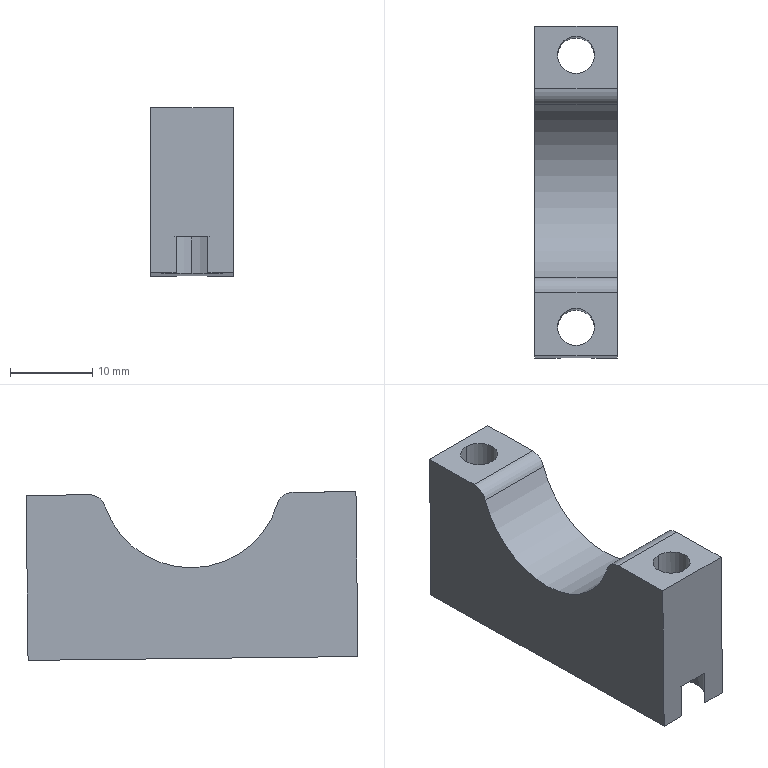Component | SolidWorks | 10-1111-1 | 1 solid | 19 faces | box 10 x 40.23 x 20.46 mm | volume 5601 mm3 | cylinder 10 | plane 9 | commonest cylinder face diameters 4.5 x4 8 x3 4 x2 22 x1 | material AL6061(GB)Natural Anodized
build123d program:
from build123d import *

# Parameters (mm, degrees)
SKETCH1_W                                       = 20
SKETCH1_H                                       = 10
EXTRUDE1_DEPTH                                  = 40
SKETCH2_R                                       = 11
CUT_EXTRUDE1_DEPTH                              = 46.826
M4_HEX_SOCKET_HEAD_CAP_SCREW_CBORE2_D           = 4.5
M4_HEX_SOCKET_HEAD_CAP_SCREW_CBORE2_CBORE_D     = 8
M4_HEX_SOCKET_HEAD_CAP_SCREW_CBORE2_CBORE_DEPTH = 4.4
FILLET1_R                                       = 2


with BuildPart() as part:
    # Sketch1 → Extrude1 (new body)
    with BuildSketch(Plane.XY):
        with Locations((10, 5)):
            Rectangle(SKETCH1_W, SKETCH1_H)
    extrude(amount=EXTRUDE1_DEPTH)

    # Sketch2 → Cut-Extrude1 (cut, through all)
    with BuildSketch(Plane(origin=(0, 10, 0), x_dir=(1, 0, 0), z_dir=(0, 1, 0))):
        with Locations((-2, -20)):
            Circle(SKETCH2_R)
    extrude(amount=-CUT_EXTRUDE1_DEPTH, mode=Mode.SUBTRACT)

    # M4 Hex Socket Head Cap Screw CBORE2 (through all)
    with Locations(Plane(origin=(20, 5, 36.5), x_dir=(0, 0, 1), z_dir=(1, 0, 0))):
        with Locations((0, 0), (-33, 0)):
            CounterBoreHole(M4_HEX_SOCKET_HEAD_CAP_SCREW_CBORE2_D / 2, M4_HEX_SOCKET_HEAD_CAP_SCREW_CBORE2_CBORE_D / 2, M4_HEX_SOCKET_HEAD_CAP_SCREW_CBORE2_CBORE_DEPTH)

    # Fillet1
    fillet1_edges = [part.edges().sort_by_distance(p)[0] for p in [
        (0, 5, 9.183),
        (0, 5, 30.817),
    ]]
    fillet(fillet1_edges, radius=FILLET1_R)


solid = part.part

# Placed as in the assembly
solid = solid.moved(Location((105, -75.022, -76.768), (-90.665, 0, 90)))
STEP:
#1=CARTESIAN_POINT('',(3.937,-2.904,-3.023));
#2=VERTEX_POINT('',#1);
#3=CARTESIAN_POINT('',(3.937,-2.727,-3.025));
#4=VERTEX_POINT('',#3);
#5=CARTESIAN_POINT('',(3.937,-2.816,-3.024));
#6=DIRECTION('',(0.,-0.0116,-0.9999));
#7=DIRECTION('',(0.,0.9999,-0.0116));
#8=AXIS2_PLACEMENT_3D('',#5,#6,#7);
#9=CIRCLE('',#8,0.08858);
#10=EDGE_CURVE('',#2,#4,#9,.T.);
#11=ORIENTED_EDGE('',*,*,#10,.F.);
#12=CARTESIAN_POINT('',(3.937,-2.912,-3.637));
#13=VERTEX_POINT('',#12);
#14=CARTESIAN_POINT('',(3.937,-2.914,-3.81));
#15=DIRECTION('',(0.,-0.0116,-0.9999));
#16=VECTOR('',#15,39.37);
#17=LINE('',#14,#16);
#18=EDGE_CURVE('',#2,#13,#17,.T.);
#19=ORIENTED_EDGE('',*,*,#18,.T.);
#20=CARTESIAN_POINT('',(3.937,-2.734,-3.639));
#21=VERTEX_POINT('',#20);
#22=CARTESIAN_POINT('',(3.937,-2.823,-3.638));
#23=DIRECTION('',(0.,-0.0116,-0.9999));
#24=DIRECTION('',(0.,0.9999,-0.0116));
#25=AXIS2_PLACEMENT_3D('',#22,#23,#24);
#26=CIRCLE('',#25,0.08858);
#27=EDGE_CURVE('',#13,#21,#26,.T.);
#28=ORIENTED_EDGE('',*,*,#27,.T.);
#29=CARTESIAN_POINT('',(3.937,-2.736,-3.812));
#30=DIRECTION('',(0.,-0.0116,-0.9999));
#31=VECTOR('',#30,39.37);
#32=LINE('',#29,#31);
#33=EDGE_CURVE('',#4,#21,#32,.T.);
#34=ORIENTED_EDGE('',*,*,#33,.F.);
#35=EDGE_LOOP('',(#11,#19,#28,#34));
#36=FACE_OUTER_BOUND('',#35,.T.);
#37=CARTESIAN_POINT('',(3.937,-2.825,-3.811));
#38=DIRECTION('',(0.,-0.0116,-0.9999));
#39=DIRECTION('',(0.,0.9999,-0.0116));
#40=AXIS2_PLACEMENT_3D('',#37,#38,#39);
#41=CYLINDRICAL_SURFACE('',#40,0.08858);
#42=ADVANCED_FACE('',(#36),#41,.F.);
#43=CARTESIAN_POINT('',(3.937,-2.665,-3.64));
#44=VERTEX_POINT('',#43);
#45=CARTESIAN_POINT('',(4.013,-2.961,-3.636));
#46=VERTEX_POINT('',#45);
#47=CARTESIAN_POINT('',(3.937,-2.823,-3.638));
#48=DIRECTION('',(0.,-0.0116,-0.9999));
#49=DIRECTION('',(0.,0.9999,-0.0116));
#50=AXIS2_PLACEMENT_3D('',#47,#48,#49);
#51=CIRCLE('',#50,0.1575);
#52=EDGE_CURVE('',#44,#46,#51,.T.);
#53=ORIENTED_EDGE('',*,*,#52,.F.);
#54=CARTESIAN_POINT('',(3.937,-2.667,-3.813));
#55=VERTEX_POINT('',#54);
#56=CARTESIAN_POINT('',(3.937,-2.667,-3.813));
#57=DIRECTION('',(0.,-0.0116,-0.9999));
#58=VECTOR('',#57,39.37);
#59=LINE('',#56,#58);
#60=EDGE_CURVE('',#44,#55,#59,.T.);
#61=ORIENTED_EDGE('',*,*,#60,.T.);
#62=CARTESIAN_POINT('',(4.013,-2.963,-3.81));
#63=VERTEX_POINT('',#62);
#64=CARTESIAN_POINT('',(3.937,-2.825,-3.811));
#65=DIRECTION('',(0.,-0.0116,-0.9999));
#66=DIRECTION('',(0.,0.9999,-0.0116));
#67=AXIS2_PLACEMENT_3D('',#64,#65,#66);
#68=CIRCLE('',#67,0.1575);
#69=EDGE_CURVE('',#55,#63,#68,.T.);
#70=ORIENTED_EDGE('',*,*,#69,.T.);
#71=CARTESIAN_POINT('',(4.013,-2.963,-3.81));
#72=DIRECTION('',(0.,-0.0116,-0.9999));
#73=VECTOR('',#72,39.37);
#74=LINE('',#71,#73);
#75=EDGE_CURVE('',#46,#63,#74,.T.);
#76=ORIENTED_EDGE('',*,*,#75,.F.);
#77=EDGE_LOOP('',(#53,#61,#70,#76));
#78=FACE_OUTER_BOUND('',#77,.T.);
#79=CARTESIAN_POINT('',(3.937,-2.825,-3.811));
#80=DIRECTION('',(0.,-0.0116,-0.9999));
#81=DIRECTION('',(0.,0.9999,-0.0116));
#82=AXIS2_PLACEMENT_3D('',#79,#80,#81);
#83=CYLINDRICAL_SURFACE('',#82,0.1575);
#84=ADVANCED_FACE('',(#78),#83,.F.);
#85=CARTESIAN_POINT('',(3.937,-1.605,-3.038));
#86=VERTEX_POINT('',#85);
#87=CARTESIAN_POINT('',(3.937,-1.428,-3.04));
#88=VERTEX_POINT('',#87);
#89=CARTESIAN_POINT('',(3.937,-1.517,-3.039));
#90=DIRECTION('',(0.,-0.0116,-0.9999));
#91=DIRECTION('',(0.,0.9999,-0.0116));
#92=AXIS2_PLACEMENT_3D('',#89,#90,#91);
#93=CIRCLE('',#92,0.08858);
#94=EDGE_CURVE('',#86,#88,#93,.T.);
#95=ORIENTED_EDGE('',*,*,#94,.F.);
#96=CARTESIAN_POINT('',(3.937,-1.612,-3.652));
#97=VERTEX_POINT('',#96);
#98=CARTESIAN_POINT('',(3.937,-1.614,-3.825));
#99=DIRECTION('',(0.,-0.0116,-0.9999));
#100=VECTOR('',#99,39.37);
#101=LINE('',#98,#100);
#102=EDGE_CURVE('',#86,#97,#101,.T.);
#103=ORIENTED_EDGE('',*,*,#102,.T.);
#104=CARTESIAN_POINT('',(3.937,-1.435,-3.654));
#105=VERTEX_POINT('',#104);
#106=CARTESIAN_POINT('',(3.937,-1.524,-3.653));
#107=DIRECTION('',(0.,-0.0116,-0.9999));
#108=DIRECTION('',(0.,0.9999,-0.0116));
#109=AXIS2_PLACEMENT_3D('',#106,#107,#108);
#110=CIRCLE('',#109,0.08858);
#111=EDGE_CURVE('',#97,#105,#110,.T.);
#112=ORIENTED_EDGE('',*,*,#111,.T.);
#113=CARTESIAN_POINT('',(3.937,-1.437,-3.827));
#114=DIRECTION('',(0.,-0.0116,-0.9999));
#115=VECTOR('',#114,39.37);
#116=LINE('',#113,#115);
#117=EDGE_CURVE('',#88,#105,#116,.T.);
#118=ORIENTED_EDGE('',*,*,#117,.F.);
#119=EDGE_LOOP('',(#95,#103,#112,#118));
#120=FACE_OUTER_BOUND('',#119,.T.);
#121=CARTESIAN_POINT('',(3.937,-1.526,-3.826));
#122=DIRECTION('',(0.,-0.0116,-0.9999));
#123=DIRECTION('',(0.,0.9999,-0.0116));
#124=AXIS2_PLACEMENT_3D('',#121,#122,#123);
#125=CYLINDRICAL_SURFACE('',#124,0.08858);
#126=ADVANCED_FACE('',(#120),#125,.F.);
#127=CARTESIAN_POINT('',(3.937,-1.517,-3.039));
#128=DIRECTION('',(0.,-0.0116,-0.9999));
#129=DIRECTION('',(0.,0.9999,-0.0116));
#130=AXIS2_PLACEMENT_3D('',#127,#128,#129);
#131=CIRCLE('',#130,0.08858);
#132=EDGE_CURVE('',#88,#86,#131,.T.);
#133=ORIENTED_EDGE('',*,*,#132,.T.);
#134=ORIENTED_EDGE('',*,*,#94,.T.);
#135=EDGE_LOOP('',(#133,#134));
#136=FACE_BOUND('',#135,.T.);
#137=CARTESIAN_POINT('',(3.74,-1.679,-3.037));
#138=VERTEX_POINT('',#137);
#139=CARTESIAN_POINT('',(3.74,-1.379,-3.041));
#140=VERTEX_POINT('',#139);
#141=CARTESIAN_POINT('',(3.74,-2.954,-3.022));
#142=DIRECTION('',(0.,0.9999,-0.0116));
#143=VECTOR('',#142,39.37);
#144=LINE('',#141,#143);
#145=EDGE_CURVE('',#138,#140,#144,.T.);
#146=ORIENTED_EDGE('',*,*,#145,.F.);
#147=CARTESIAN_POINT('',(4.134,-1.679,-3.037));
#148=VERTEX_POINT('',#147);
#149=CARTESIAN_POINT('',(3.74,-1.679,-3.037));
#150=DIRECTION('',(1.,-0.,0.));
#151=VECTOR('',#150,39.37);
#152=LINE('',#149,#151);
#153=EDGE_CURVE('',#138,#148,#152,.T.);
#154=ORIENTED_EDGE('',*,*,#153,.T.);
#155=CARTESIAN_POINT('',(4.134,-1.379,-3.041));
#156=VERTEX_POINT('',#155);
#157=CARTESIAN_POINT('',(4.134,-2.954,-3.022));
#158=DIRECTION('',(0.,0.9999,-0.0116));
#159=VECTOR('',#158,39.37);
#160=LINE('',#157,#159);
#161=EDGE_CURVE('',#148,#156,#160,.T.);
#162=ORIENTED_EDGE('',*,*,#161,.T.);
#163=CARTESIAN_POINT('',(3.74,-1.379,-3.041));
#164=DIRECTION('',(-1.,0.,-0.));
#165=VECTOR('',#164,39.37);
#166=LINE('',#163,#165);
#167=EDGE_CURVE('',#156,#140,#166,.T.);
#168=ORIENTED_EDGE('',*,*,#167,.T.);
#169=EDGE_LOOP('',(#146,#154,#162,#168));
#170=FACE_OUTER_BOUND('',#169,.T.);
#171=CARTESIAN_POINT('',(3.74,-2.954,-3.022));
#172=DIRECTION('',(0.,-0.0116,-0.9999));
#173=DIRECTION('',(0.,0.9999,-0.0116));
#174=AXIS2_PLACEMENT_3D('',#171,#172,#173);
#175=PLANE('',#174);
#176=ADVANCED_FACE('',(#136,#170),#175,.F.);
#177=CARTESIAN_POINT('',(3.937,-2.816,-3.024));
#178=DIRECTION('',(0.,-0.0116,-0.9999));
#179=DIRECTION('',(0.,0.9999,-0.0116));
#180=AXIS2_PLACEMENT_3D('',#177,#178,#179);
#181=CIRCLE('',#180,0.08858);
#182=EDGE_CURVE('',#4,#2,#181,.T.);
#183=ORIENTED_EDGE('',*,*,#182,.T.);
#184=ORIENTED_EDGE('',*,*,#10,.T.);
#185=EDGE_LOOP('',(#183,#184));
#186=FACE_BOUND('',#185,.T.);
#187=CARTESIAN_POINT('',(4.134,-2.954,-3.022));
#188=VERTEX_POINT('',#187);
#189=CARTESIAN_POINT('',(4.134,-2.653,-3.026));
#190=VERTEX_POINT('',#189);
#191=CARTESIAN_POINT('',(4.134,-2.954,-3.022));
#192=DIRECTION('',(0.,0.9999,-0.0116));
#193=VECTOR('',#192,39.37);
#194=LINE('',#191,#193);
#195=EDGE_CURVE('',#188,#190,#194,.T.);
#196=ORIENTED_EDGE('',*,*,#195,.T.);
#197=CARTESIAN_POINT('',(3.74,-2.653,-3.026));
#198=VERTEX_POINT('',#197);
#199=CARTESIAN_POINT('',(3.74,-2.653,-3.026));
#200=DIRECTION('',(-1.,0.,-0.));
#201=VECTOR('',#200,39.37);
#202=LINE('',#199,#201);
#203=EDGE_CURVE('',#190,#198,#202,.T.);
#204=ORIENTED_EDGE('',*,*,#203,.T.);
#205=CARTESIAN_POINT('',(3.74,-2.954,-3.022));
#206=VERTEX_POINT('',#205);
#207=CARTESIAN_POINT('',(3.74,-2.954,-3.022));
#208=DIRECTION('',(0.,0.9999,-0.0116));
#209=VECTOR('',#208,39.37);
#210=LINE('',#207,#209);
#211=EDGE_CURVE('',#206,#198,#210,.T.);
#212=ORIENTED_EDGE('',*,*,#211,.F.);
#213=CARTESIAN_POINT('',(3.74,-2.954,-3.022));
#214=DIRECTION('',(-1.,0.,-0.));
#215=VECTOR('',#214,39.37);
#216=LINE('',#213,#215);
#217=EDGE_CURVE('',#188,#206,#216,.T.);
#218=ORIENTED_EDGE('',*,*,#217,.F.);
#219=EDGE_LOOP('',(#196,#204,#212,#218));
#220=FACE_OUTER_BOUND('',#219,.T.);
#221=CARTESIAN_POINT('',(3.74,-2.954,-3.022));
#222=DIRECTION('',(0.,-0.0116,-0.9999));
#223=DIRECTION('',(0.,0.9999,-0.0116));
#224=AXIS2_PLACEMENT_3D('',#221,#222,#223);
#225=PLANE('',#224);
#226=ADVANCED_FACE('',(#186,#220),#225,.F.);
#227=ORIENTED_EDGE('',*,*,#211,.T.);
#228=CARTESIAN_POINT('',(3.74,-2.579,-3.081));
#229=VERTEX_POINT('',#228);
#230=CARTESIAN_POINT('',(3.74,-2.654,-3.105));
#231=DIRECTION('',(-1.,0.,-0.));
#232=DIRECTION('',(0.,-0.9999,0.0116));
#233=AXIS2_PLACEMENT_3D('',#230,#231,#232);
#234=CIRCLE('',#233,0.07874);
#235=EDGE_CURVE('',#198,#229,#234,.T.);
#236=ORIENTED_EDGE('',*,*,#235,.T.);
#237=CARTESIAN_POINT('',(3.74,-1.755,-3.091));
#238=VERTEX_POINT('',#237);
#239=CARTESIAN_POINT('',(3.74,-2.165,-2.953));
#240=DIRECTION('',(1.,-0.,0.));
#241=DIRECTION('',(0.,-0.9999,0.0116));
#242=AXIS2_PLACEMENT_3D('',#239,#240,#241);
#243=CIRCLE('',#242,0.4331);
#244=EDGE_CURVE('',#229,#238,#243,.T.);
#245=ORIENTED_EDGE('',*,*,#244,.T.);
#246=CARTESIAN_POINT('',(3.74,-1.68,-3.116));
#247=DIRECTION('',(-1.,0.,-0.));
#248=DIRECTION('',(0.,-0.9999,0.0116));
#249=AXIS2_PLACEMENT_3D('',#246,#247,#248);
#250=CIRCLE('',#249,0.07874);
#251=EDGE_CURVE('',#238,#138,#250,.T.);
#252=ORIENTED_EDGE('',*,*,#251,.T.);
#253=ORIENTED_EDGE('',*,*,#145,.T.);
#254=CARTESIAN_POINT('',(3.74,-1.388,-3.828));
#255=VERTEX_POINT('',#254);
#256=CARTESIAN_POINT('',(3.74,-1.379,-3.041));
#257=DIRECTION('',(0.,-0.0116,-0.9999));
#258=VECTOR('',#257,39.37);
#259=LINE('',#256,#258);
#260=EDGE_CURVE('',#140,#255,#259,.T.);
#261=ORIENTED_EDGE('',*,*,#260,.T.);
#262=CARTESIAN_POINT('',(3.74,-2.963,-3.81));
#263=VERTEX_POINT('',#262);
#264=CARTESIAN_POINT('',(3.74,-2.963,-3.81));
#265=DIRECTION('',(0.,0.9999,-0.0116));
#266=VECTOR('',#265,39.37);
#267=LINE('',#264,#266);
#268=EDGE_CURVE('',#263,#255,#267,.T.);
#269=ORIENTED_EDGE('',*,*,#268,.F.);
#270=CARTESIAN_POINT('',(3.74,-2.954,-3.022));
#271=DIRECTION('',(0.,-0.0116,-0.9999));
#272=VECTOR('',#271,39.37);
#273=LINE('',#270,#272);
#274=EDGE_CURVE('',#206,#263,#273,.T.);
#275=ORIENTED_EDGE('',*,*,#274,.F.);
#276=EDGE_LOOP('',(#227,#236,#245,#252,#253,#261,#269,#275));
#277=FACE_OUTER_BOUND('',#276,.T.);
#278=CARTESIAN_POINT('',(3.74,-2.954,-3.022));
#279=DIRECTION('',(1.,-0.,0.));
#280=DIRECTION('',(-0.,-0.9999,0.0116));
#281=AXIS2_PLACEMENT_3D('',#278,#279,#280);
#282=PLANE('',#281);
#283=ADVANCED_FACE('',(#277),#282,.F.);
#284=CARTESIAN_POINT('',(4.134,-2.963,-3.81));
#285=VERTEX_POINT('',#284);
#286=CARTESIAN_POINT('',(3.74,-2.963,-3.81));
#287=DIRECTION('',(1.,-0.,0.));
#288=VECTOR('',#287,39.37);
#289=LINE('',#286,#288);
#290=EDGE_CURVE('',#63,#285,#289,.T.);
#291=ORIENTED_EDGE('',*,*,#290,.F.);
#292=ORIENTED_EDGE('',*,*,#69,.F.);
#293=CARTESIAN_POINT('',(3.861,-2.963,-3.81));
#294=VERTEX_POINT('',#293);
#295=CARTESIAN_POINT('',(3.937,-2.825,-3.811));
#296=DIRECTION('',(0.,-0.0116,-0.9999));
#297=DIRECTION('',(0.,0.9999,-0.0116));
#298=AXIS2_PLACEMENT_3D('',#295,#296,#297);
#299=CIRCLE('',#298,0.1575);
#300=EDGE_CURVE('',#294,#55,#299,.T.);
#301=ORIENTED_EDGE('',*,*,#300,.F.);
#302=CARTESIAN_POINT('',(3.74,-2.963,-3.81));
#303=DIRECTION('',(1.,-0.,0.));
#304=VECTOR('',#303,39.37);
#305=LINE('',#302,#304);
#306=EDGE_CURVE('',#263,#294,#305,.T.);
#307=ORIENTED_EDGE('',*,*,#306,.F.);
#308=ORIENTED_EDGE('',*,*,#268,.T.);
#309=CARTESIAN_POINT('',(3.861,-1.388,-3.828));
#310=VERTEX_POINT('',#309);
#311=CARTESIAN_POINT('',(3.74,-1.388,-3.828));
#312=DIRECTION('',(1.,-0.,0.));
#313=VECTOR('',#312,39.37);
#314=LINE('',#311,#313);
#315=EDGE_CURVE('',#255,#310,#314,.T.);
#316=ORIENTED_EDGE('',*,*,#315,.T.);
#317=CARTESIAN_POINT('',(4.013,-1.388,-3.828));
#318=VERTEX_POINT('',#317);
#319=CARTESIAN_POINT('',(3.937,-1.526,-3.826));
#320=DIRECTION('',(0.,-0.0116,-0.9999));
#321=DIRECTION('',(0.,0.9999,-0.0116));
#322=AXIS2_PLACEMENT_3D('',#319,#320,#321);
#323=CIRCLE('',#322,0.1575);
#324=EDGE_CURVE('',#318,#310,#323,.T.);
#325=ORIENTED_EDGE('',*,*,#324,.F.);
#326=CARTESIAN_POINT('',(4.134,-1.388,-3.828));
#327=VERTEX_POINT('',#326);
#328=CARTESIAN_POINT('',(3.74,-1.388,-3.828));
#329=DIRECTION('',(1.,-0.,0.));
#330=VECTOR('',#329,39.37);
#331=LINE('',#328,#330);
#332=EDGE_CURVE('',#318,#327,#331,.T.);
#333=ORIENTED_EDGE('',*,*,#332,.T.);
#334=CARTESIAN_POINT('',(4.134,-2.963,-3.81));
#335=DIRECTION('',(0.,0.9999,-0.0116));
#336=VECTOR('',#335,39.37);
#337=LINE('',#334,#336);
#338=EDGE_CURVE('',#285,#327,#337,.T.);
#339=ORIENTED_EDGE('',*,*,#338,.F.);
#340=EDGE_LOOP('',(#291,#292,#301,#307,#308,#316,#325,#333,#339));
#341=FACE_OUTER_BOUND('',#340,.T.);
#342=CARTESIAN_POINT('',(3.74,-2.963,-3.81));
#343=DIRECTION('',(-0.,0.0116,0.9999));
#344=DIRECTION('',(-0.,-0.9999,0.0116));
#345=AXIS2_PLACEMENT_3D('',#342,#343,#344);
#346=PLANE('',#345);
#347=ADVANCED_FACE('',(#341),#346,.F.);
#348=CARTESIAN_POINT('',(4.134,-2.579,-3.081));
#349=VERTEX_POINT('',#348);
#350=CARTESIAN_POINT('',(4.134,-1.755,-3.091));
#351=VERTEX_POINT('',#350);
#352=CARTESIAN_POINT('',(4.134,-2.165,-2.953));
#353=DIRECTION('',(1.,-0.,0.));
#354=DIRECTION('',(0.,-0.9999,0.0116));
#355=AXIS2_PLACEMENT_3D('',#352,#353,#354);
#356=CIRCLE('',#355,0.4331);
#357=EDGE_CURVE('',#349,#351,#356,.T.);
#358=ORIENTED_EDGE('',*,*,#357,.F.);
#359=CARTESIAN_POINT('',(4.134,-2.654,-3.105));
#360=DIRECTION('',(1.,-0.,0.));
#361=DIRECTION('',(0.,0.9999,-0.0116));
#362=AXIS2_PLACEMENT_3D('',#359,#360,#361);
#363=CIRCLE('',#362,0.07874);
#364=EDGE_CURVE('',#349,#190,#363,.T.);
#365=ORIENTED_EDGE('',*,*,#364,.T.);
#366=ORIENTED_EDGE('',*,*,#195,.F.);
#367=CARTESIAN_POINT('',(4.134,-2.954,-3.022));
#368=DIRECTION('',(-0.,0.0116,0.9999));
#369=VECTOR('',#368,39.37);
#370=LINE('',#367,#369);
#371=EDGE_CURVE('',#285,#188,#370,.T.);
#372=ORIENTED_EDGE('',*,*,#371,.F.);
#373=ORIENTED_EDGE('',*,*,#338,.T.);
#374=CARTESIAN_POINT('',(4.134,-1.379,-3.041));
#375=DIRECTION('',(-0.,0.0116,0.9999));
#376=VECTOR('',#375,39.37);
#377=LINE('',#374,#376);
#378=EDGE_CURVE('',#327,#156,#377,.T.);
#379=ORIENTED_EDGE('',*,*,#378,.T.);
#380=ORIENTED_EDGE('',*,*,#161,.F.);
#381=CARTESIAN_POINT('',(4.134,-1.68,-3.116));
#382=DIRECTION('',(1.,-0.,0.));
#383=DIRECTION('',(0.,0.9999,-0.0116));
#384=AXIS2_PLACEMENT_3D('',#381,#382,#383);
#385=CIRCLE('',#384,0.07874);
#386=EDGE_CURVE('',#148,#351,#385,.T.);
#387=ORIENTED_EDGE('',*,*,#386,.T.);
#388=EDGE_LOOP('',(#358,#365,#366,#372,#373,#379,#380,#387));
#389=FACE_OUTER_BOUND('',#388,.T.);
#390=CARTESIAN_POINT('',(4.134,-2.954,-3.022));
#391=DIRECTION('',(-1.,0.,-0.));
#392=DIRECTION('',(0.,0.9999,-0.0116));
#393=AXIS2_PLACEMENT_3D('',#390,#391,#392);
#394=PLANE('',#393);
#395=ADVANCED_FACE('',(#389),#394,.F.);
#396=CARTESIAN_POINT('',(3.861,-2.961,-3.636));
#397=VERTEX_POINT('',#396);
#398=CARTESIAN_POINT('',(4.134,-2.961,-3.636));
#399=DIRECTION('',(1.,-0.,0.));
#400=VECTOR('',#399,39.37);
#401=LINE('',#398,#400);
#402=EDGE_CURVE('',#397,#46,#401,.T.);
#403=ORIENTED_EDGE('',*,*,#402,.T.);
#404=ORIENTED_EDGE('',*,*,#75,.T.);
#405=ORIENTED_EDGE('',*,*,#290,.T.);
#406=ORIENTED_EDGE('',*,*,#371,.T.);
#407=ORIENTED_EDGE('',*,*,#217,.T.);
#408=ORIENTED_EDGE('',*,*,#274,.T.);
#409=ORIENTED_EDGE('',*,*,#306,.T.);
#410=CARTESIAN_POINT('',(3.861,-2.963,-3.81));
#411=DIRECTION('',(-0.,0.0116,0.9999));
#412=VECTOR('',#411,39.37);
#413=LINE('',#410,#412);
#414=EDGE_CURVE('',#294,#397,#413,.T.);
#415=ORIENTED_EDGE('',*,*,#414,.T.);
#416=EDGE_LOOP('',(#403,#404,#405,#406,#407,#408,#409,#415));
#417=FACE_OUTER_BOUND('',#416,.T.);
#418=CARTESIAN_POINT('',(4.134,-2.954,-3.022));
#419=DIRECTION('',(0.,0.9999,-0.0116));
#420=DIRECTION('',(-0.,0.0116,0.9999));
#421=AXIS2_PLACEMENT_3D('',#418,#419,#420);
#422=PLANE('',#421);
#423=ADVANCED_FACE('',(#417),#422,.F.);
#424=CARTESIAN_POINT('',(4.013,-1.386,-3.655));
#425=VERTEX_POINT('',#424);
#426=CARTESIAN_POINT('',(4.013,-1.388,-3.828));
#427=DIRECTION('',(0.,-0.0116,-0.9999));
#428=VECTOR('',#427,39.37);
#429=LINE('',#426,#428);
#430=EDGE_CURVE('',#425,#318,#429,.T.);
#431=ORIENTED_EDGE('',*,*,#430,.F.);
#432=CARTESIAN_POINT('',(3.861,-1.386,-3.655));
#433=VERTEX_POINT('',#432);
#434=CARTESIAN_POINT('',(4.134,-1.386,-3.655));
#435=DIRECTION('',(1.,-0.,0.));
#436=VECTOR('',#435,39.37);
#437=LINE('',#434,#436);
#438=EDGE_CURVE('',#433,#425,#437,.T.);
#439=ORIENTED_EDGE('',*,*,#438,.F.);
#440=CARTESIAN_POINT('',(3.861,-1.388,-3.828));
#441=DIRECTION('',(-0.,0.0116,0.9999));
#442=VECTOR('',#441,39.37);
#443=LINE('',#440,#442);
#444=EDGE_CURVE('',#310,#433,#443,.T.);
#445=ORIENTED_EDGE('',*,*,#444,.F.);
#446=ORIENTED_EDGE('',*,*,#315,.F.);
#447=ORIENTED_EDGE('',*,*,#260,.F.);
#448=ORIENTED_EDGE('',*,*,#167,.F.);
#449=ORIENTED_EDGE('',*,*,#378,.F.);
#450=ORIENTED_EDGE('',*,*,#332,.F.);
#451=EDGE_LOOP('',(#431,#439,#445,#446,#447,#448,#449,#450));
#452=FACE_OUTER_BOUND('',#451,.T.);
#453=CARTESIAN_POINT('',(4.134,-1.379,-3.041));
#454=DIRECTION('',(0.,0.9999,-0.0116));
#455=DIRECTION('',(-0.,0.0116,0.9999));
#456=AXIS2_PLACEMENT_3D('',#453,#454,#455);
#457=PLANE('',#456);
#458=ADVANCED_FACE('',(#452),#457,.T.);
#459=ORIENTED_EDGE('',*,*,#244,.F.);
#460=CARTESIAN_POINT('',(3.74,-2.579,-3.081));
#461=DIRECTION('',(1.,-0.,0.));
#462=VECTOR('',#461,39.37);
#463=LINE('',#460,#462);
#464=EDGE_CURVE('',#229,#349,#463,.T.);
#465=ORIENTED_EDGE('',*,*,#464,.T.);
#466=ORIENTED_EDGE('',*,*,#357,.T.);
#467=CARTESIAN_POINT('',(3.74,-1.755,-3.091));
#468=DIRECTION('',(-1.,0.,-0.));
#469=VECTOR('',#468,39.37);
#470=LINE('',#467,#469);
#471=EDGE_CURVE('',#351,#238,#470,.T.);
#472=ORIENTED_EDGE('',*,*,#471,.T.);
#473=EDGE_LOOP('',(#459,#465,#466,#472));
#474=FACE_OUTER_BOUND('',#473,.T.);
#475=CARTESIAN_POINT('',(3.74,-2.165,-2.953));
#476=DIRECTION('',(1.,-0.,0.));
#477=DIRECTION('',(0.,-0.9999,0.0116));
#478=AXIS2_PLACEMENT_3D('',#475,#476,#477);
#479=CYLINDRICAL_SURFACE('',#478,0.4331);
#480=ADVANCED_FACE('',(#474),#479,.F.);
#481=ORIENTED_EDGE('',*,*,#102,.F.);
#482=ORIENTED_EDGE('',*,*,#132,.F.);
#483=ORIENTED_EDGE('',*,*,#117,.T.);
#484=CARTESIAN_POINT('',(3.937,-1.524,-3.653));
#485=DIRECTION('',(0.,-0.0116,-0.9999));
#486=DIRECTION('',(0.,0.9999,-0.0116));
#487=AXIS2_PLACEMENT_3D('',#484,#485,#486);
#488=CIRCLE('',#487,0.08858);
#489=EDGE_CURVE('',#105,#97,#488,.T.);
#490=ORIENTED_EDGE('',*,*,#489,.T.);
#491=EDGE_LOOP('',(#481,#482,#483,#490));
#492=FACE_OUTER_BOUND('',#491,.T.);
#493=CARTESIAN_POINT('',(3.937,-1.526,-3.826));
#494=DIRECTION('',(0.,-0.0116,-0.9999));
#495=DIRECTION('',(0.,0.9999,-0.0116));
#496=AXIS2_PLACEMENT_3D('',#493,#494,#495);
#497=CYLINDRICAL_SURFACE('',#496,0.08858);
#498=ADVANCED_FACE('',(#492),#497,.F.);
#499=ORIENTED_EDGE('',*,*,#438,.T.);
#500=CARTESIAN_POINT('',(3.937,-1.524,-3.653));
#501=DIRECTION('',(0.,-0.0116,-0.9999));
#502=DIRECTION('',(0.,0.9999,-0.0116));
#503=AXIS2_PLACEMENT_3D('',#500,#501,#502);
#504=CIRCLE('',#503,0.1575);
#505=EDGE_CURVE('',#425,#433,#504,.T.);
#506=ORIENTED_EDGE('',*,*,#505,.T.);
#507=EDGE_LOOP('',(#499,#506));
#508=FACE_OUTER_BOUND('',#507,.T.);
#509=ORIENTED_EDGE('',*,*,#489,.F.);
#510=ORIENTED_EDGE('',*,*,#111,.F.);
#511=EDGE_LOOP('',(#509,#510));
#512=FACE_BOUND('',#511,.T.);
#513=CARTESIAN_POINT('',(4.026,-1.524,-3.653));
#514=DIRECTION('',(-0.,0.0116,0.9999));
#515=DIRECTION('',(-0.,-0.9999,0.0116));
#516=AXIS2_PLACEMENT_3D('',#513,#514,#515);
#517=PLANE('',#516);
#518=ADVANCED_FACE('',(#508,#512),#517,.F.);
#519=ORIENTED_EDGE('',*,*,#430,.T.);
#520=ORIENTED_EDGE('',*,*,#324,.T.);
#521=ORIENTED_EDGE('',*,*,#444,.T.);
#522=ORIENTED_EDGE('',*,*,#505,.F.);
#523=EDGE_LOOP('',(#519,#520,#521,#522));
#524=FACE_OUTER_BOUND('',#523,.T.);
#525=CARTESIAN_POINT('',(3.937,-1.526,-3.826));
#526=DIRECTION('',(0.,-0.0116,-0.9999));
#527=DIRECTION('',(0.,0.9999,-0.0116));
#528=AXIS2_PLACEMENT_3D('',#525,#526,#527);
#529=CYLINDRICAL_SURFACE('',#528,0.1575);
#530=ADVANCED_FACE('',(#524),#529,.F.);
#531=CARTESIAN_POINT('',(3.937,-2.823,-3.638));
#532=DIRECTION('',(0.,-0.0116,-0.9999));
#533=DIRECTION('',(0.,0.9999,-0.0116));
#534=AXIS2_PLACEMENT_3D('',#531,#532,#533);
#535=CIRCLE('',#534,0.08858);
#536=EDGE_CURVE('',#21,#13,#535,.T.);
#537=ORIENTED_EDGE('',*,*,#536,.F.);
#538=ORIENTED_EDGE('',*,*,#27,.F.);
#539=EDGE_LOOP('',(#537,#538));
#540=FACE_BOUND('',#539,.T.);
#541=CARTESIAN_POINT('',(3.937,-2.823,-3.638));
#542=DIRECTION('',(0.,-0.0116,-0.9999));
#543=DIRECTION('',(0.,0.9999,-0.0116));
#544=AXIS2_PLACEMENT_3D('',#541,#542,#543);
#545=CIRCLE('',#544,0.1575);
#546=EDGE_CURVE('',#397,#44,#545,.T.);
#547=ORIENTED_EDGE('',*,*,#546,.T.);
#548=ORIENTED_EDGE('',*,*,#52,.T.);
#549=ORIENTED_EDGE('',*,*,#402,.F.);
#550=EDGE_LOOP('',(#547,#548,#549));
#551=FACE_OUTER_BOUND('',#550,.T.);
#552=CARTESIAN_POINT('',(4.026,-2.823,-3.638));
#553=DIRECTION('',(-0.,0.0116,0.9999));
#554=DIRECTION('',(-0.,-0.9999,0.0116));
#555=AXIS2_PLACEMENT_3D('',#552,#553,#554);
#556=PLANE('',#555);
#557=ADVANCED_FACE('',(#540,#551),#556,.F.);
#558=ORIENTED_EDGE('',*,*,#60,.F.);
#559=ORIENTED_EDGE('',*,*,#546,.F.);
#560=ORIENTED_EDGE('',*,*,#414,.F.);
#561=ORIENTED_EDGE('',*,*,#300,.T.);
#562=EDGE_LOOP('',(#558,#559,#560,#561));
#563=FACE_OUTER_BOUND('',#562,.T.);
#564=CARTESIAN_POINT('',(3.937,-2.825,-3.811));
#565=DIRECTION('',(0.,-0.0116,-0.9999));
#566=DIRECTION('',(0.,0.9999,-0.0116));
#567=AXIS2_PLACEMENT_3D('',#564,#565,#566);
#568=CYLINDRICAL_SURFACE('',#567,0.1575);
#569=ADVANCED_FACE('',(#563),#568,.F.);
#570=ORIENTED_EDGE('',*,*,#18,.F.);
#571=ORIENTED_EDGE('',*,*,#182,.F.);
#572=ORIENTED_EDGE('',*,*,#33,.T.);
#573=ORIENTED_EDGE('',*,*,#536,.T.);
#574=EDGE_LOOP('',(#570,#571,#572,#573));
#575=FACE_OUTER_BOUND('',#574,.T.);
#576=CARTESIAN_POINT('',(3.937,-2.825,-3.811));
#577=DIRECTION('',(0.,-0.0116,-0.9999));
#578=DIRECTION('',(0.,0.9999,-0.0116));
#579=AXIS2_PLACEMENT_3D('',#576,#577,#578);
#580=CYLINDRICAL_SURFACE('',#579,0.08858);
#581=ADVANCED_FACE('',(#575),#580,.F.);
#582=ORIENTED_EDGE('',*,*,#364,.F.);
#583=ORIENTED_EDGE('',*,*,#464,.F.);
#584=ORIENTED_EDGE('',*,*,#235,.F.);
#585=ORIENTED_EDGE('',*,*,#203,.F.);
#586=EDGE_LOOP('',(#582,#583,#584,#585));
#587=FACE_OUTER_BOUND('',#586,.T.);
#588=CARTESIAN_POINT('',(3.74,-2.654,-3.105));
#589=DIRECTION('',(1.,-0.,0.));
#590=DIRECTION('',(0.,-0.9999,0.0116));
#591=AXIS2_PLACEMENT_3D('',#588,#589,#590);
#592=CYLINDRICAL_SURFACE('',#591,0.07874);
#593=ADVANCED_FACE('',(#587),#592,.T.);
#594=ORIENTED_EDGE('',*,*,#251,.F.);
#595=ORIENTED_EDGE('',*,*,#471,.F.);
#596=ORIENTED_EDGE('',*,*,#386,.F.);
#597=ORIENTED_EDGE('',*,*,#153,.F.);
#598=EDGE_LOOP('',(#594,#595,#596,#597));
#599=FACE_OUTER_BOUND('',#598,.T.);
#600=CARTESIAN_POINT('',(3.74,-1.68,-3.116));
#601=DIRECTION('',(1.,-0.,0.));
#602=DIRECTION('',(0.,-0.9999,0.0116));
#603=AXIS2_PLACEMENT_3D('',#600,#601,#602);
#604=CYLINDRICAL_SURFACE('',#603,0.07874);
#605=ADVANCED_FACE('',(#599),#604,.T.);
#606=CLOSED_SHELL('',(#42,#84,#126,#176,#226,#283,#347,#395,#423,#458,#480,#498,#518,#530,#557,#569,#581,#593,#605));
#607=MANIFOLD_SOLID_BREP('',#606);
#608=CARTESIAN_POINT('',(0.,0.,0.));
#609=DIRECTION('',(0.,0.,1.));
#610=DIRECTION('',(1.,0.,0.));
#611=AXIS2_PLACEMENT_3D('',#608,#609,#610);
#612=(LENGTH_UNIT()NAMED_UNIT(*)SI_UNIT($,.METRE.));
#613=LENGTH_MEASURE_WITH_UNIT(LENGTH_MEASURE(0.0254),#612);
#614=DIMENSIONAL_EXPONENTS(1.,0.,0.,0.,0.,0.,0.);
#615=(CONVERSION_BASED_UNIT('',#613)LENGTH_UNIT()NAMED_UNIT(#614));
#616=UNCERTAINTY_MEASURE_WITH_UNIT(LENGTH_MEASURE(0.00001),#615,'','');
#617=(NAMED_UNIT(*)PLANE_ANGLE_UNIT()SI_UNIT($,.RADIAN.));
#618=(NAMED_UNIT(*)SI_UNIT($,.STERADIAN.)SOLID_ANGLE_UNIT());
#619=(GEOMETRIC_REPRESENTATION_CONTEXT(3)GLOBAL_UNCERTAINTY_ASSIGNED_CONTEXT((#616))GLOBAL_UNIT_ASSIGNED_CONTEXT((#615,#617,#618))REPRESENTATION_CONTEXT('',''));
#620=ADVANCED_BREP_SHAPE_REPRESENTATION('',(#607,#611),#619);
#621=COLOUR_RGB('',0.7922,0.8196,0.9333);
#622=FILL_AREA_STYLE_COLOUR('',#621);
#623=FILL_AREA_STYLE('',(#622));
#624=SURFACE_STYLE_FILL_AREA(#623);
#625=SURFACE_SIDE_STYLE('',(#624));
#626=SURFACE_STYLE_USAGE(.BOTH.,#625);
#627=PRESENTATION_STYLE_ASSIGNMENT((#626));
#628=STYLED_ITEM('',(#627),#607);
#629=PRESENTATION_LAYER_ASSIGNMENT('','',(#628));
#630=(LENGTH_UNIT()NAMED_UNIT(*)SI_UNIT($,.METRE.));
#631=LENGTH_MEASURE_WITH_UNIT(LENGTH_MEASURE(0.0254),#630);
#632=DIMENSIONAL_EXPONENTS(1.,0.,0.,0.,0.,0.,0.);
#633=(CONVERSION_BASED_UNIT('',#631)LENGTH_UNIT()NAMED_UNIT(#632));
#634=UNCERTAINTY_MEASURE_WITH_UNIT(LENGTH_MEASURE(0.00001),#633,'','');
#635=(NAMED_UNIT(*)PLANE_ANGLE_UNIT()SI_UNIT($,.RADIAN.));
#636=(NAMED_UNIT(*)SI_UNIT($,.STERADIAN.)SOLID_ANGLE_UNIT());
#637=(GEOMETRIC_REPRESENTATION_CONTEXT(3)GLOBAL_UNCERTAINTY_ASSIGNED_CONTEXT((#634))GLOBAL_UNIT_ASSIGNED_CONTEXT((#633,#635,#636))REPRESENTATION_CONTEXT('',''));
#638=MECHANICAL_DESIGN_GEOMETRIC_PRESENTATION_REPRESENTATION('',(#628),#637);